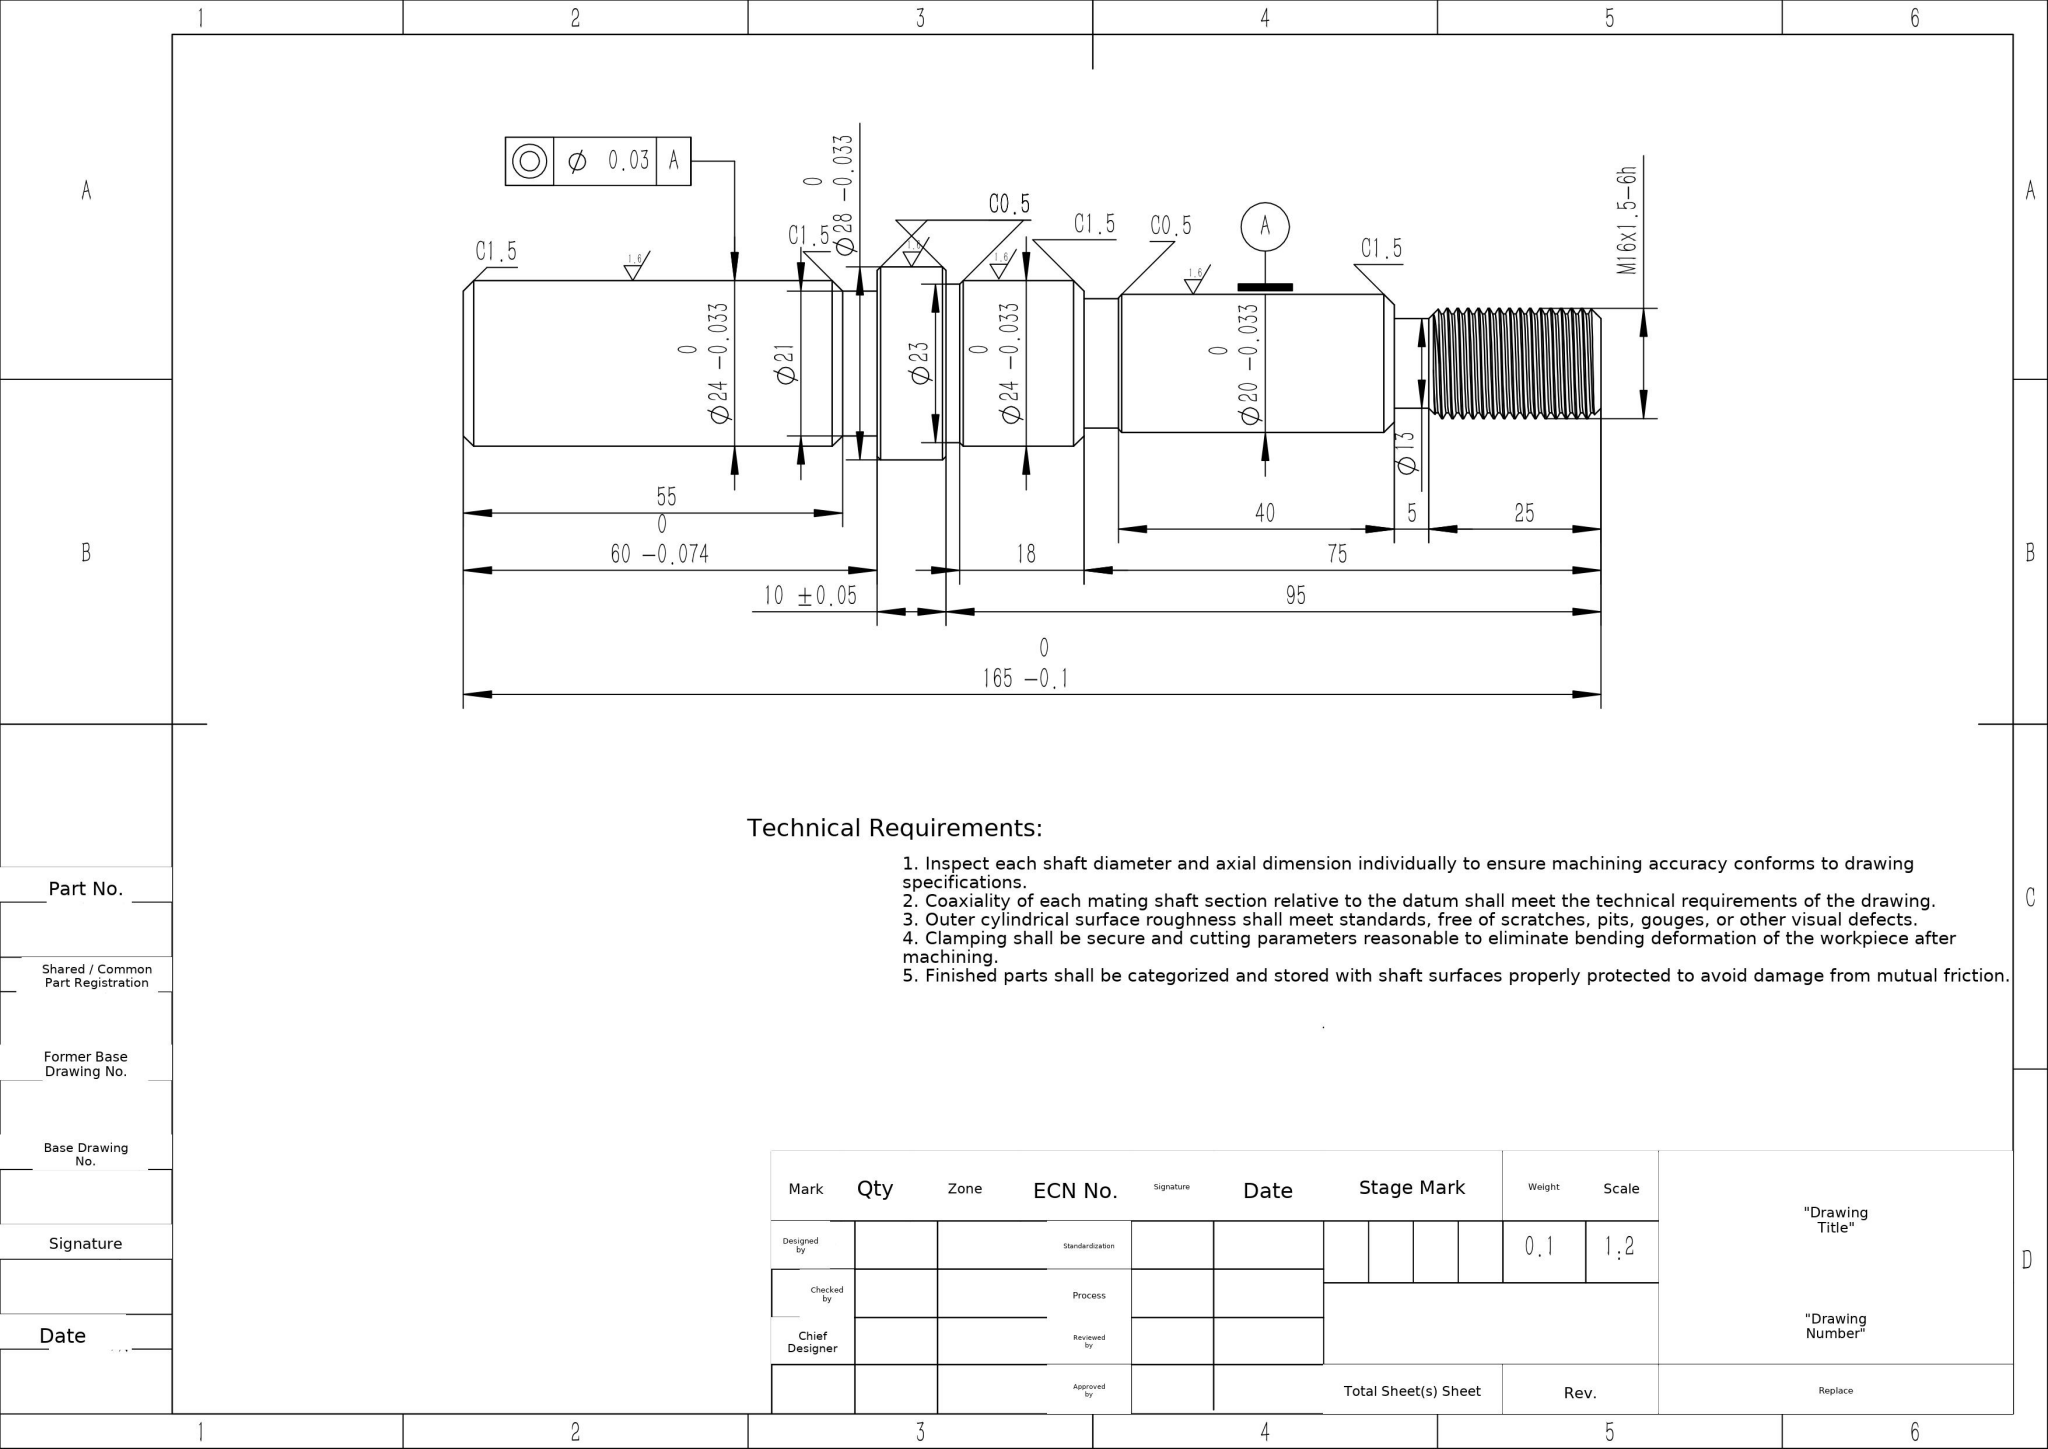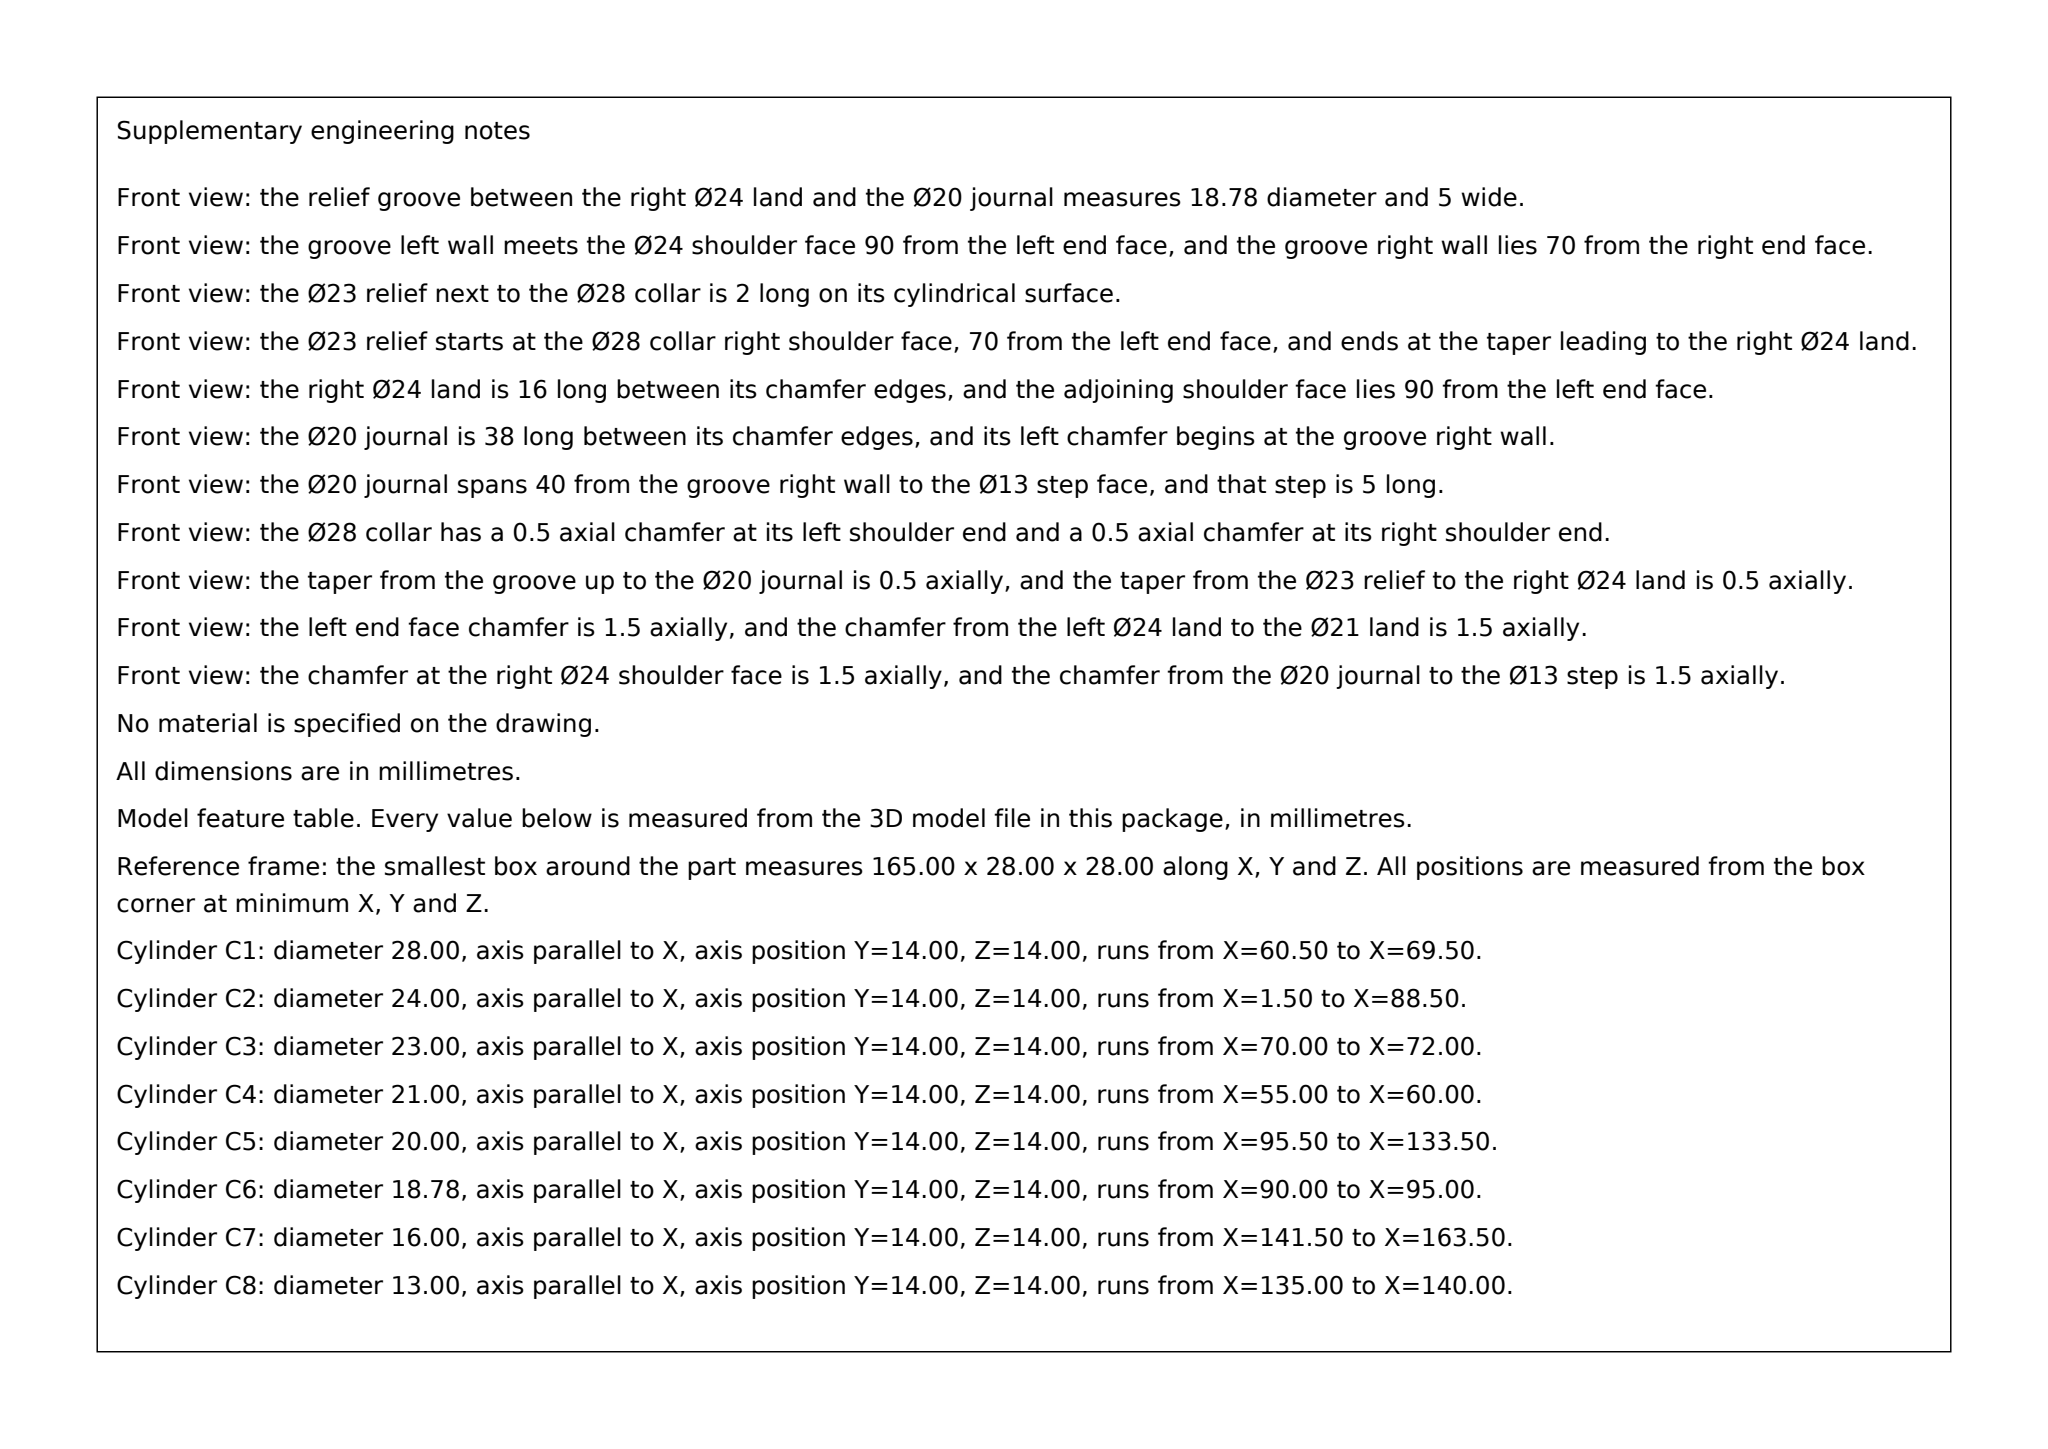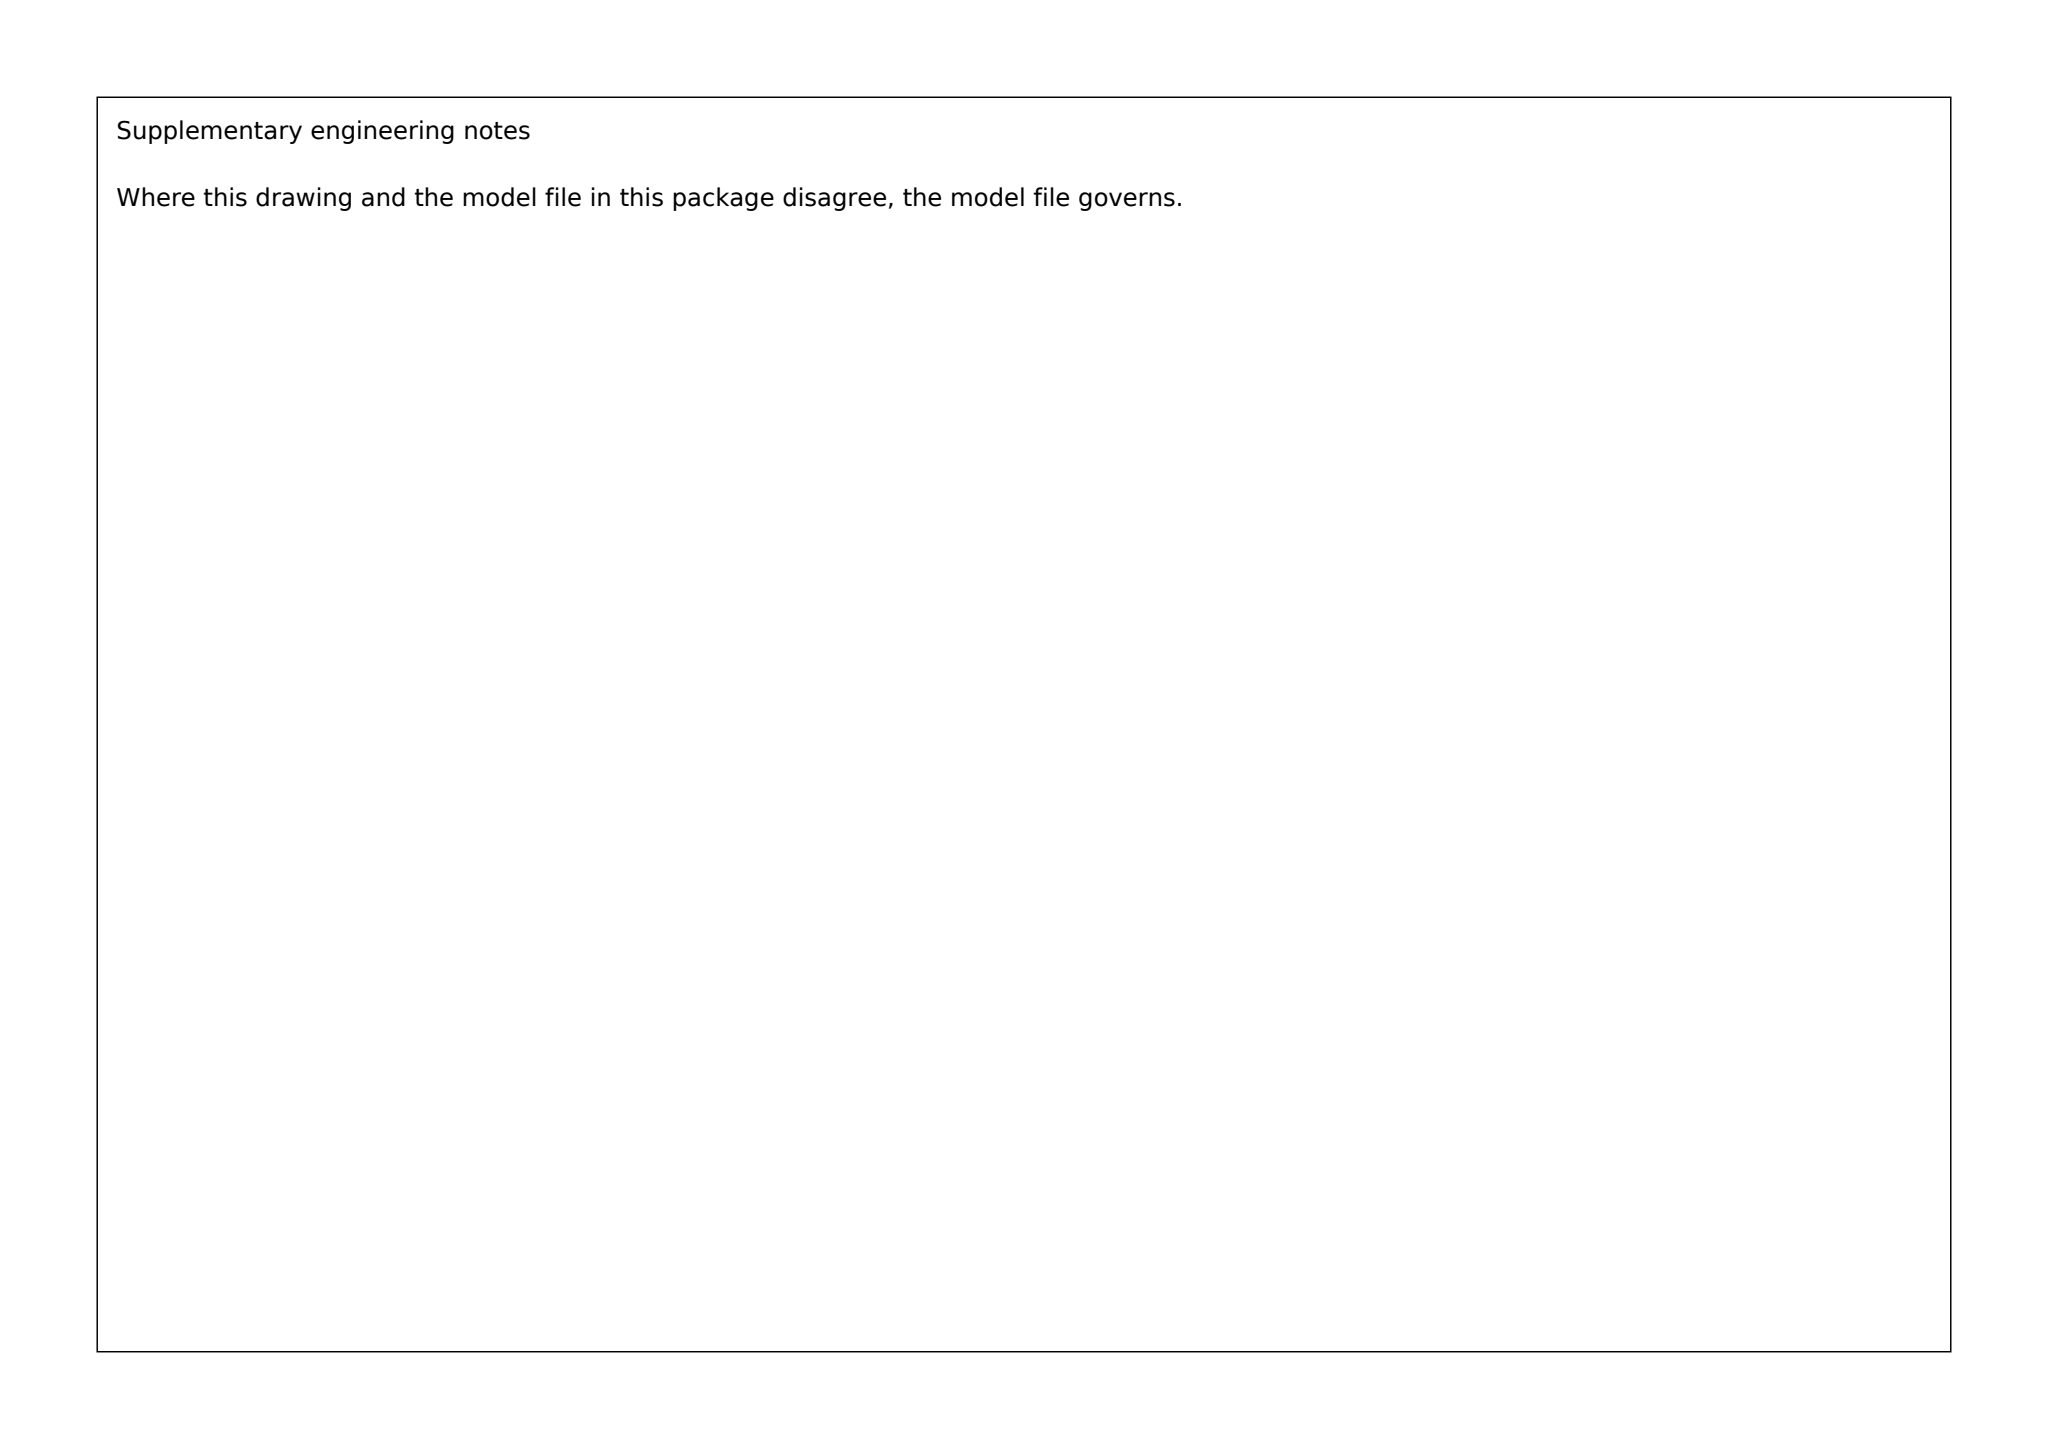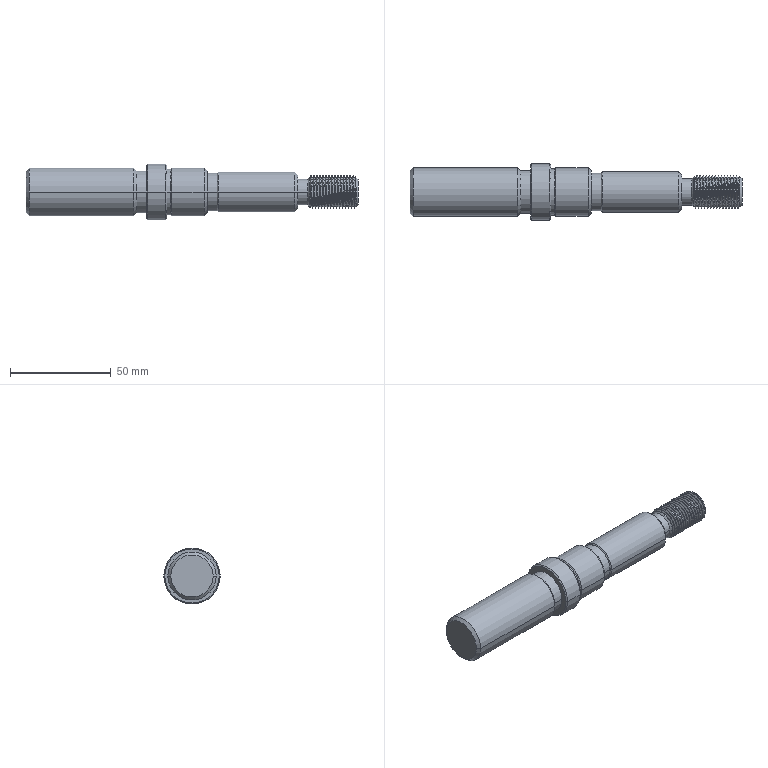Part | SolidWorks | mm | 1 solid | 82 faces | box 165 x 28 x 28 mm | volume 59855 mm3 | cylinder 46 | cone 21 | plane 8 | spline 7 | commonest cylinder face diameters 16 x30 24 x4 13 x2 20 x2 18.78 x2 23 x2 28 x2 21 x2
Drawing notes:
RELIEF GROOVE Ø18.8 (18.78) x 5 WIDE, LEFT WALL 90 FROM LEFT END FACE (GROOVE SPANS 90 TO 95). | from the solid: cylinder dia 18.78, axis x, length 5.0; axis planes x=90.0 and x=95.0 (5 mm apart)
C1.5 x 45 DEG LEAD-IN CHAMFER (Ø16 TO Ø13) AT FREE RIGHT-HAND END OF THREAD, AT x=165 END FACE. | from the solid: cones 90 deg included at ref dia 16.0 and 13.0 at thread end; plane x=165.0
ALL DIMENSIONS IN MILLIMETRES (mm). | from the solid: STEP model units mm, bbox_xyz 165.0 x 28.0 x 28.0